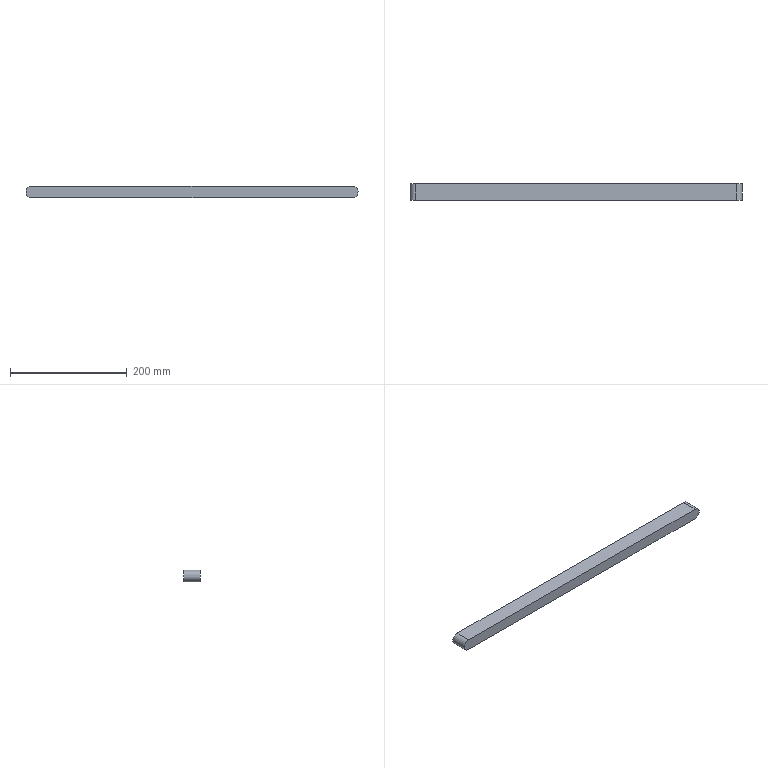Component | NX | MAIN_SHAFT_KEY | 1 solid | 6 faces | box 570 x 28 x 20 mm | volume 316796 mm3 | plane 4 | cylinder 2 | commonest cylinder face diameters 20 x2
STEP:
#1=CARTESIAN_POINT('',(0.,0.,0.));
#2=DIRECTION('',(0.,0.,1.));
#3=DIRECTION('',(1.,0.,0.));
#4=AXIS2_PLACEMENT_3D('',#1,#2,#3);
#5=CARTESIAN_POINT('',(149.458,-1128.882,829.997));
#6=VERTEX_POINT('',#5);
#7=CARTESIAN_POINT('',(699.458,-1128.882,829.997));
#8=VERTEX_POINT('',#7);
#9=CARTESIAN_POINT('',(149.458,-1128.882,829.997));
#10=DIRECTION('',(1.,0.,0.));
#11=VECTOR('',#10,1.);
#12=LINE('',#9,#11);
#13=CARTESIAN_POINT('',(149.458,-1100.882,829.997));
#14=DIRECTION('',(0.,0.,-1.));
#15=DIRECTION('',(0.,1.,0.));
#16=AXIS2_PLACEMENT_3D('',#13,#14,#15);
#17=PLANE('',#16);
#18=CARTESIAN_POINT('',(-28.,0.));
#19=DIRECTION('',(0.,1.));
#20=VECTOR('',#19,1.);
#21=LINE('',#18,#20);
#22=(GEOMETRIC_REPRESENTATION_CONTEXT(2)PARAMETRIC_REPRESENTATION_CONTEXT()REPRESENTATION_CONTEXT('',''));
#23=DEFINITIONAL_REPRESENTATION('',(#21),#22);
#24=PCURVE('',#17,#23);
#25=CARTESIAN_POINT('',(699.458,-1128.882,839.997));
#26=DIRECTION('',(0.,-1.,0.));
#27=DIRECTION('',(-1.,0.,0.));
#28=AXIS2_PLACEMENT_3D('',#25,#26,#27);
#29=PLANE('',#28);
#30=CARTESIAN_POINT('',(550.,10.));
#31=DIRECTION('',(-1.,0.));
#32=VECTOR('',#31,1.);
#33=LINE('',#30,#32);
#34=(GEOMETRIC_REPRESENTATION_CONTEXT(2)PARAMETRIC_REPRESENTATION_CONTEXT()REPRESENTATION_CONTEXT('',''));
#35=DEFINITIONAL_REPRESENTATION('',(#33),#34);
#36=PCURVE('',#29,#35);
#37=SURFACE_CURVE('',#12,(#24,#36),.PCURVE_S1.);
#38=EDGE_CURVE('',#6,#8,#37,.T.);
#39=ORIENTED_EDGE('',*,*,#38,.F.);
#40=CARTESIAN_POINT('',(149.458,-1100.882,829.997));
#41=VERTEX_POINT('',#40);
#42=CARTESIAN_POINT('',(149.458,-1100.882,829.997));
#43=DIRECTION('',(0.,-1.,0.));
#44=VECTOR('',#43,1.);
#45=LINE('',#42,#44);
#46=CARTESIAN_POINT('',(0.,0.));
#47=DIRECTION('',(-1.,0.));
#48=VECTOR('',#47,1.);
#49=LINE('',#46,#48);
#50=(GEOMETRIC_REPRESENTATION_CONTEXT(2)PARAMETRIC_REPRESENTATION_CONTEXT()REPRESENTATION_CONTEXT('',''));
#51=DEFINITIONAL_REPRESENTATION('',(#49),#50);
#52=PCURVE('',#17,#51);
#53=CARTESIAN_POINT('',(149.458,-1100.882,839.997));
#54=DIRECTION('',(0.,-1.,0.));
#55=DIRECTION('',(-1.,0.,0.));
#56=AXIS2_PLACEMENT_3D('',#53,#54,#55);
#57=CYLINDRICAL_SURFACE('',#56,10.);
#58=CARTESIAN_POINT('',(7.854,0.));
#59=DIRECTION('',(0.,1.));
#60=VECTOR('',#59,1.);
#61=LINE('',#58,#60);
#62=(GEOMETRIC_REPRESENTATION_CONTEXT(2)PARAMETRIC_REPRESENTATION_CONTEXT()REPRESENTATION_CONTEXT('',''));
#63=DEFINITIONAL_REPRESENTATION('',(#61),#62);
#64=PCURVE('',#57,#63);
#65=SURFACE_CURVE('',#45,(#52,#64),.PCURVE_S1.);
#66=EDGE_CURVE('',#41,#6,#65,.T.);
#67=ORIENTED_EDGE('',*,*,#66,.F.);
#68=CARTESIAN_POINT('',(699.458,-1100.882,829.997));
#69=VERTEX_POINT('',#68);
#70=CARTESIAN_POINT('',(149.458,-1100.882,829.997));
#71=DIRECTION('',(1.,0.,0.));
#72=VECTOR('',#71,1.);
#73=LINE('',#70,#72);
#74=CARTESIAN_POINT('',(0.,0.));
#75=DIRECTION('',(0.,1.));
#76=VECTOR('',#75,1.);
#77=LINE('',#74,#76);
#78=(GEOMETRIC_REPRESENTATION_CONTEXT(2)PARAMETRIC_REPRESENTATION_CONTEXT()REPRESENTATION_CONTEXT('',''));
#79=DEFINITIONAL_REPRESENTATION('',(#77),#78);
#80=PCURVE('',#17,#79);
#81=CARTESIAN_POINT('',(699.458,-1100.882,839.997));
#82=DIRECTION('',(0.,-1.,0.));
#83=DIRECTION('',(-1.,0.,0.));
#84=AXIS2_PLACEMENT_3D('',#81,#82,#83);
#85=PLANE('',#84);
#86=CARTESIAN_POINT('',(550.,10.));
#87=DIRECTION('',(-1.,0.));
#88=VECTOR('',#87,1.);
#89=LINE('',#86,#88);
#90=(GEOMETRIC_REPRESENTATION_CONTEXT(2)PARAMETRIC_REPRESENTATION_CONTEXT()REPRESENTATION_CONTEXT('',''));
#91=DEFINITIONAL_REPRESENTATION('',(#89),#90);
#92=PCURVE('',#85,#91);
#93=SURFACE_CURVE('',#73,(#80,#92),.PCURVE_S1.);
#94=EDGE_CURVE('',#41,#69,#93,.T.);
#95=ORIENTED_EDGE('',*,*,#94,.T.);
#96=CARTESIAN_POINT('',(699.458,-1100.882,829.997));
#97=DIRECTION('',(0.,-1.,0.));
#98=VECTOR('',#97,1.);
#99=LINE('',#96,#98);
#100=CARTESIAN_POINT('',(0.,550.));
#101=DIRECTION('',(-1.,0.));
#102=VECTOR('',#101,1.);
#103=LINE('',#100,#102);
#104=(GEOMETRIC_REPRESENTATION_CONTEXT(2)PARAMETRIC_REPRESENTATION_CONTEXT()REPRESENTATION_CONTEXT('',''));
#105=DEFINITIONAL_REPRESENTATION('',(#103),#104);
#106=PCURVE('',#17,#105);
#107=CARTESIAN_POINT('',(699.458,-1100.882,839.997));
#108=DIRECTION('',(0.,-1.,0.));
#109=DIRECTION('',(-1.,0.,0.));
#110=AXIS2_PLACEMENT_3D('',#107,#108,#109);
#111=CYLINDRICAL_SURFACE('',#110,10.);
#112=CARTESIAN_POINT('',(1.571,0.));
#113=DIRECTION('',(0.,1.));
#114=VECTOR('',#113,1.);
#115=LINE('',#112,#114);
#116=(GEOMETRIC_REPRESENTATION_CONTEXT(2)PARAMETRIC_REPRESENTATION_CONTEXT()REPRESENTATION_CONTEXT('',''));
#117=DEFINITIONAL_REPRESENTATION('',(#115),#116);
#118=PCURVE('',#111,#117);
#119=SURFACE_CURVE('',#99,(#106,#118),.PCURVE_S1.);
#120=EDGE_CURVE('',#69,#8,#119,.T.);
#121=ORIENTED_EDGE('',*,*,#120,.T.);
#122=EDGE_LOOP('',(#39,#67,#95,#121));
#123=FACE_BOUND('',#122,.T.);
#124=ADVANCED_FACE('',(#123),#17,.T.);
#125=CARTESIAN_POINT('',(699.458,-1128.882,849.997));
#126=VERTEX_POINT('',#125);
#127=CARTESIAN_POINT('',(699.458,-1128.882,839.997));
#128=DIRECTION('',(0.,-1.,0.));
#129=DIRECTION('',(1.,0.,0.));
#130=AXIS2_PLACEMENT_3D('',#127,#128,#129);
#131=CIRCLE('',#130,10.);
#132=CARTESIAN_POINT('',(-3.142,28.));
#133=DIRECTION('',(1.,0.));
#134=VECTOR('',#133,1.);
#135=LINE('',#132,#134);
#136=(GEOMETRIC_REPRESENTATION_CONTEXT(2)PARAMETRIC_REPRESENTATION_CONTEXT()REPRESENTATION_CONTEXT('',''));
#137=DEFINITIONAL_REPRESENTATION('',(#135),#136);
#138=PCURVE('',#111,#137);
#139=CARTESIAN_POINT('',(0.,0.));
#140=DIRECTION('',(-1.,0.));
#141=AXIS2_PLACEMENT_2D('',#139,#140);
#142=CIRCLE('',#141,10.);
#143=(GEOMETRIC_REPRESENTATION_CONTEXT(2)PARAMETRIC_REPRESENTATION_CONTEXT()REPRESENTATION_CONTEXT('',''));
#144=DEFINITIONAL_REPRESENTATION('',(#142),#143);
#145=PCURVE('',#29,#144);
#146=SURFACE_CURVE('',#131,(#138,#145),.PCURVE_S1.);
#147=EDGE_CURVE('',#8,#126,#146,.T.);
#148=ORIENTED_EDGE('',*,*,#147,.F.);
#149=ORIENTED_EDGE('',*,*,#120,.F.);
#150=CARTESIAN_POINT('',(699.458,-1100.882,849.997));
#151=VERTEX_POINT('',#150);
#152=CARTESIAN_POINT('',(699.458,-1100.882,839.997));
#153=DIRECTION('',(0.,-1.,0.));
#154=DIRECTION('',(1.,0.,0.));
#155=AXIS2_PLACEMENT_3D('',#152,#153,#154);
#156=CIRCLE('',#155,10.);
#157=CARTESIAN_POINT('',(-3.142,0.));
#158=DIRECTION('',(1.,0.));
#159=VECTOR('',#158,1.);
#160=LINE('',#157,#159);
#161=(GEOMETRIC_REPRESENTATION_CONTEXT(2)PARAMETRIC_REPRESENTATION_CONTEXT()REPRESENTATION_CONTEXT('',''));
#162=DEFINITIONAL_REPRESENTATION('',(#160),#161);
#163=PCURVE('',#111,#162);
#164=CARTESIAN_POINT('',(0.,0.));
#165=DIRECTION('',(-1.,0.));
#166=AXIS2_PLACEMENT_2D('',#164,#165);
#167=CIRCLE('',#166,10.);
#168=(GEOMETRIC_REPRESENTATION_CONTEXT(2)PARAMETRIC_REPRESENTATION_CONTEXT()REPRESENTATION_CONTEXT('',''));
#169=DEFINITIONAL_REPRESENTATION('',(#167),#168);
#170=PCURVE('',#85,#169);
#171=SURFACE_CURVE('',#156,(#163,#170),.PCURVE_S1.);
#172=EDGE_CURVE('',#69,#151,#171,.T.);
#173=ORIENTED_EDGE('',*,*,#172,.T.);
#174=CARTESIAN_POINT('',(699.458,-1100.882,849.997));
#175=DIRECTION('',(0.,-1.,0.));
#176=VECTOR('',#175,1.);
#177=LINE('',#174,#176);
#178=CARTESIAN_POINT('',(4.712,0.));
#179=DIRECTION('',(0.,1.));
#180=VECTOR('',#179,1.);
#181=LINE('',#178,#180);
#182=(GEOMETRIC_REPRESENTATION_CONTEXT(2)PARAMETRIC_REPRESENTATION_CONTEXT()REPRESENTATION_CONTEXT('',''));
#183=DEFINITIONAL_REPRESENTATION('',(#181),#182);
#184=PCURVE('',#111,#183);
#185=CARTESIAN_POINT('',(699.458,-1100.882,849.997));
#186=DIRECTION('',(0.,0.,1.));
#187=DIRECTION('',(0.,-1.,0.));
#188=AXIS2_PLACEMENT_3D('',#185,#186,#187);
#189=PLANE('',#188);
#190=CARTESIAN_POINT('',(0.,0.));
#191=DIRECTION('',(1.,0.));
#192=VECTOR('',#191,1.);
#193=LINE('',#190,#192);
#194=(GEOMETRIC_REPRESENTATION_CONTEXT(2)PARAMETRIC_REPRESENTATION_CONTEXT()REPRESENTATION_CONTEXT('',''));
#195=DEFINITIONAL_REPRESENTATION('',(#193),#194);
#196=PCURVE('',#189,#195);
#197=SURFACE_CURVE('',#177,(#184,#196),.PCURVE_S1.);
#198=EDGE_CURVE('',#151,#126,#197,.T.);
#199=ORIENTED_EDGE('',*,*,#198,.T.);
#200=EDGE_LOOP('',(#148,#149,#173,#199));
#201=FACE_BOUND('',#200,.T.);
#202=ADVANCED_FACE('',(#201),#111,.T.);
#203=CARTESIAN_POINT('',(149.458,-1128.882,849.997));
#204=VERTEX_POINT('',#203);
#205=CARTESIAN_POINT('',(699.458,-1128.882,849.997));
#206=DIRECTION('',(-1.,0.,0.));
#207=VECTOR('',#206,1.);
#208=LINE('',#205,#207);
#209=CARTESIAN_POINT('',(28.,0.));
#210=DIRECTION('',(0.,-1.));
#211=VECTOR('',#210,1.);
#212=LINE('',#209,#211);
#213=(GEOMETRIC_REPRESENTATION_CONTEXT(2)PARAMETRIC_REPRESENTATION_CONTEXT()REPRESENTATION_CONTEXT('',''));
#214=DEFINITIONAL_REPRESENTATION('',(#212),#213);
#215=PCURVE('',#189,#214);
#216=CARTESIAN_POINT('',(0.,-10.));
#217=DIRECTION('',(1.,0.));
#218=VECTOR('',#217,1.);
#219=LINE('',#216,#218);
#220=(GEOMETRIC_REPRESENTATION_CONTEXT(2)PARAMETRIC_REPRESENTATION_CONTEXT()REPRESENTATION_CONTEXT('',''));
#221=DEFINITIONAL_REPRESENTATION('',(#219),#220);
#222=PCURVE('',#29,#221);
#223=SURFACE_CURVE('',#208,(#215,#222),.PCURVE_S1.);
#224=EDGE_CURVE('',#126,#204,#223,.T.);
#225=ORIENTED_EDGE('',*,*,#224,.F.);
#226=ORIENTED_EDGE('',*,*,#198,.F.);
#227=CARTESIAN_POINT('',(149.458,-1100.882,849.997));
#228=VERTEX_POINT('',#227);
#229=CARTESIAN_POINT('',(699.458,-1100.882,849.997));
#230=DIRECTION('',(-1.,0.,0.));
#231=VECTOR('',#230,1.);
#232=LINE('',#229,#231);
#233=CARTESIAN_POINT('',(0.,0.));
#234=DIRECTION('',(0.,-1.));
#235=VECTOR('',#234,1.);
#236=LINE('',#233,#235);
#237=(GEOMETRIC_REPRESENTATION_CONTEXT(2)PARAMETRIC_REPRESENTATION_CONTEXT()REPRESENTATION_CONTEXT('',''));
#238=DEFINITIONAL_REPRESENTATION('',(#236),#237);
#239=PCURVE('',#189,#238);
#240=CARTESIAN_POINT('',(0.,-10.));
#241=DIRECTION('',(1.,0.));
#242=VECTOR('',#241,1.);
#243=LINE('',#240,#242);
#244=(GEOMETRIC_REPRESENTATION_CONTEXT(2)PARAMETRIC_REPRESENTATION_CONTEXT()REPRESENTATION_CONTEXT('',''));
#245=DEFINITIONAL_REPRESENTATION('',(#243),#244);
#246=PCURVE('',#85,#245);
#247=SURFACE_CURVE('',#232,(#239,#246),.PCURVE_S1.);
#248=EDGE_CURVE('',#151,#228,#247,.T.);
#249=ORIENTED_EDGE('',*,*,#248,.T.);
#250=CARTESIAN_POINT('',(149.458,-1100.882,849.997));
#251=DIRECTION('',(0.,-1.,0.));
#252=VECTOR('',#251,1.);
#253=LINE('',#250,#252);
#254=CARTESIAN_POINT('',(0.,-550.));
#255=DIRECTION('',(1.,0.));
#256=VECTOR('',#255,1.);
#257=LINE('',#254,#256);
#258=(GEOMETRIC_REPRESENTATION_CONTEXT(2)PARAMETRIC_REPRESENTATION_CONTEXT()REPRESENTATION_CONTEXT('',''));
#259=DEFINITIONAL_REPRESENTATION('',(#257),#258);
#260=PCURVE('',#189,#259);
#261=CARTESIAN_POINT('',(4.712,0.));
#262=DIRECTION('',(0.,1.));
#263=VECTOR('',#262,1.);
#264=LINE('',#261,#263);
#265=(GEOMETRIC_REPRESENTATION_CONTEXT(2)PARAMETRIC_REPRESENTATION_CONTEXT()REPRESENTATION_CONTEXT('',''));
#266=DEFINITIONAL_REPRESENTATION('',(#264),#265);
#267=PCURVE('',#57,#266);
#268=SURFACE_CURVE('',#253,(#260,#267),.PCURVE_S1.);
#269=EDGE_CURVE('',#228,#204,#268,.T.);
#270=ORIENTED_EDGE('',*,*,#269,.T.);
#271=EDGE_LOOP('',(#225,#226,#249,#270));
#272=FACE_BOUND('',#271,.T.);
#273=ADVANCED_FACE('',(#272),#189,.T.);
#274=CARTESIAN_POINT('',(149.458,-1128.882,839.997));
#275=DIRECTION('',(0.,-1.,0.));
#276=DIRECTION('',(1.,0.,0.));
#277=AXIS2_PLACEMENT_3D('',#274,#275,#276);
#278=CIRCLE('',#277,10.);
#279=CARTESIAN_POINT('',(3.142,28.));
#280=DIRECTION('',(1.,0.));
#281=VECTOR('',#280,1.);
#282=LINE('',#279,#281);
#283=(GEOMETRIC_REPRESENTATION_CONTEXT(2)PARAMETRIC_REPRESENTATION_CONTEXT()REPRESENTATION_CONTEXT('',''));
#284=DEFINITIONAL_REPRESENTATION('',(#282),#283);
#285=PCURVE('',#57,#284);
#286=CARTESIAN_POINT('',(550.,0.));
#287=DIRECTION('',(-1.,0.));
#288=AXIS2_PLACEMENT_2D('',#286,#287);
#289=CIRCLE('',#288,10.);
#290=(GEOMETRIC_REPRESENTATION_CONTEXT(2)PARAMETRIC_REPRESENTATION_CONTEXT()REPRESENTATION_CONTEXT('',''));
#291=DEFINITIONAL_REPRESENTATION('',(#289),#290);
#292=PCURVE('',#29,#291);
#293=SURFACE_CURVE('',#278,(#285,#292),.PCURVE_S1.);
#294=EDGE_CURVE('',#204,#6,#293,.T.);
#295=ORIENTED_EDGE('',*,*,#294,.F.);
#296=ORIENTED_EDGE('',*,*,#269,.F.);
#297=CARTESIAN_POINT('',(149.458,-1100.882,839.997));
#298=DIRECTION('',(0.,-1.,0.));
#299=DIRECTION('',(1.,0.,0.));
#300=AXIS2_PLACEMENT_3D('',#297,#298,#299);
#301=CIRCLE('',#300,10.);
#302=CARTESIAN_POINT('',(3.142,0.));
#303=DIRECTION('',(1.,0.));
#304=VECTOR('',#303,1.);
#305=LINE('',#302,#304);
#306=(GEOMETRIC_REPRESENTATION_CONTEXT(2)PARAMETRIC_REPRESENTATION_CONTEXT()REPRESENTATION_CONTEXT('',''));
#307=DEFINITIONAL_REPRESENTATION('',(#305),#306);
#308=PCURVE('',#57,#307);
#309=CARTESIAN_POINT('',(550.,0.));
#310=DIRECTION('',(-1.,0.));
#311=AXIS2_PLACEMENT_2D('',#309,#310);
#312=CIRCLE('',#311,10.);
#313=(GEOMETRIC_REPRESENTATION_CONTEXT(2)PARAMETRIC_REPRESENTATION_CONTEXT()REPRESENTATION_CONTEXT('',''));
#314=DEFINITIONAL_REPRESENTATION('',(#312),#313);
#315=PCURVE('',#85,#314);
#316=SURFACE_CURVE('',#301,(#308,#315),.PCURVE_S1.);
#317=EDGE_CURVE('',#228,#41,#316,.T.);
#318=ORIENTED_EDGE('',*,*,#317,.T.);
#319=ORIENTED_EDGE('',*,*,#66,.T.);
#320=EDGE_LOOP('',(#295,#296,#318,#319));
#321=FACE_BOUND('',#320,.T.);
#322=ADVANCED_FACE('',(#321),#57,.T.);
#323=ORIENTED_EDGE('',*,*,#94,.F.);
#324=ORIENTED_EDGE('',*,*,#317,.F.);
#325=ORIENTED_EDGE('',*,*,#248,.F.);
#326=ORIENTED_EDGE('',*,*,#172,.F.);
#327=EDGE_LOOP('',(#323,#324,#325,#326));
#328=FACE_BOUND('',#327,.T.);
#329=ADVANCED_FACE('',(#328),#85,.F.);
#330=ORIENTED_EDGE('',*,*,#38,.T.);
#331=ORIENTED_EDGE('',*,*,#147,.T.);
#332=ORIENTED_EDGE('',*,*,#224,.T.);
#333=ORIENTED_EDGE('',*,*,#294,.T.);
#334=EDGE_LOOP('',(#330,#331,#332,#333));
#335=FACE_BOUND('',#334,.T.);
#336=ADVANCED_FACE('',(#335),#29,.T.);
#337=CLOSED_SHELL('',(#124,#202,#273,#322,#329,#336));
#338=MANIFOLD_SOLID_BREP('',#337);
#339=(LENGTH_UNIT()NAMED_UNIT(*)SI_UNIT(.MILLI.,.METRE.));
#340=UNCERTAINTY_MEASURE_WITH_UNIT(LENGTH_MEASURE(0.0000001),#339,'','');
#341=(NAMED_UNIT(*)PLANE_ANGLE_UNIT()SI_UNIT($,.RADIAN.));
#342=(NAMED_UNIT(*)SI_UNIT($,.STERADIAN.)SOLID_ANGLE_UNIT());
#343=(GEOMETRIC_REPRESENTATION_CONTEXT(3)GLOBAL_UNCERTAINTY_ASSIGNED_CONTEXT((#340))GLOBAL_UNIT_ASSIGNED_CONTEXT((#339,#341,#342))REPRESENTATION_CONTEXT('',''));
#344=ADVANCED_BREP_SHAPE_REPRESENTATION('',(#4,#338),#343);